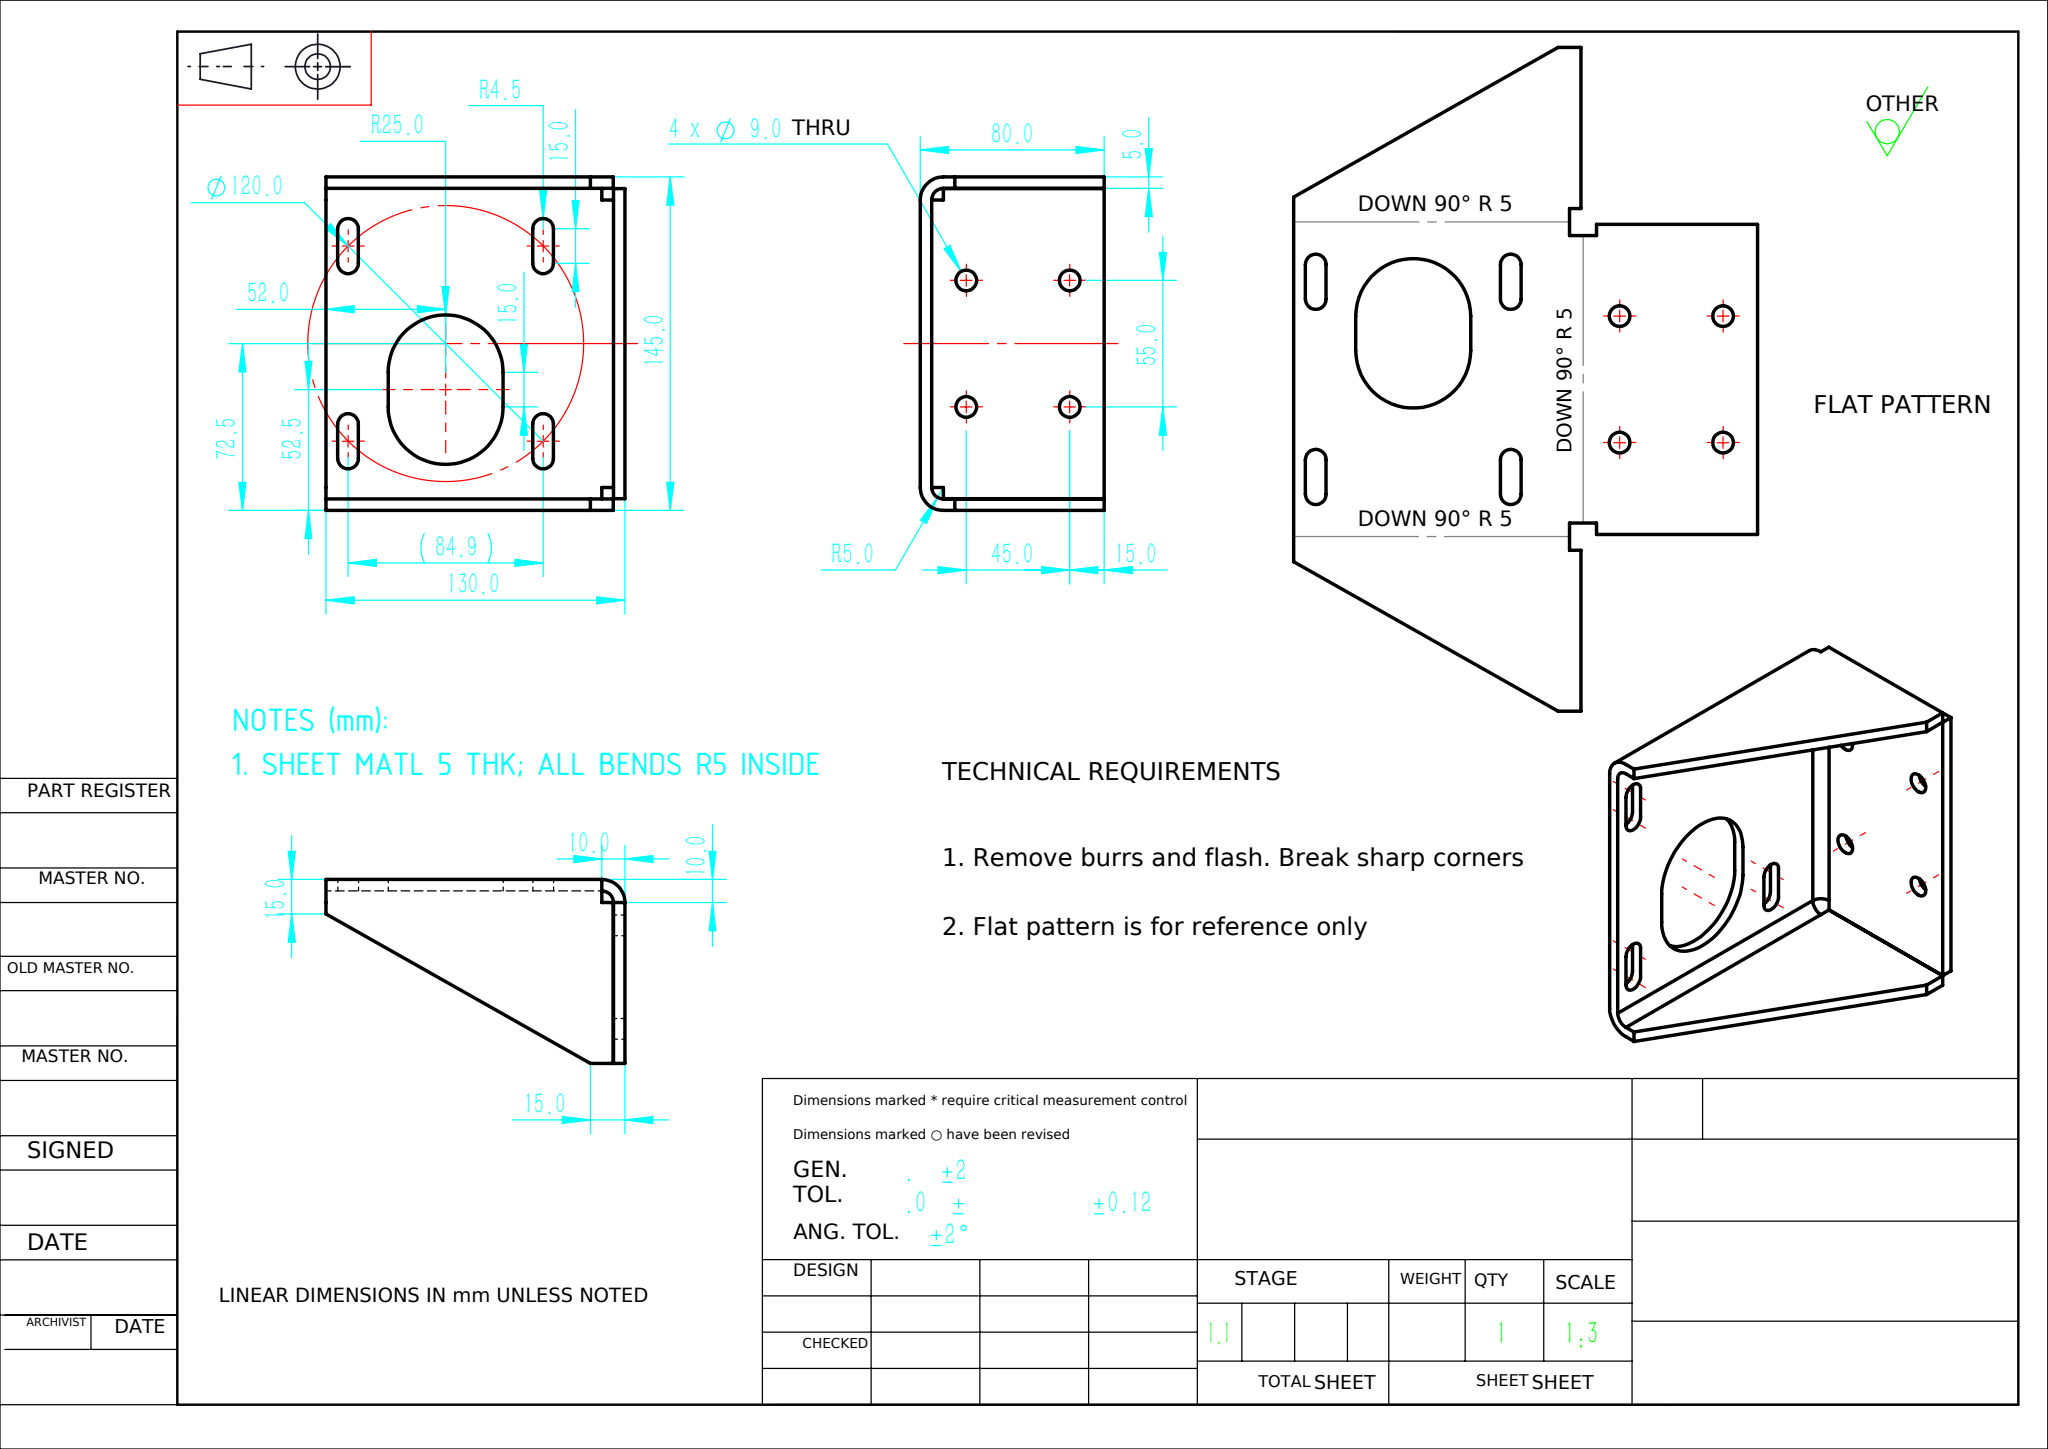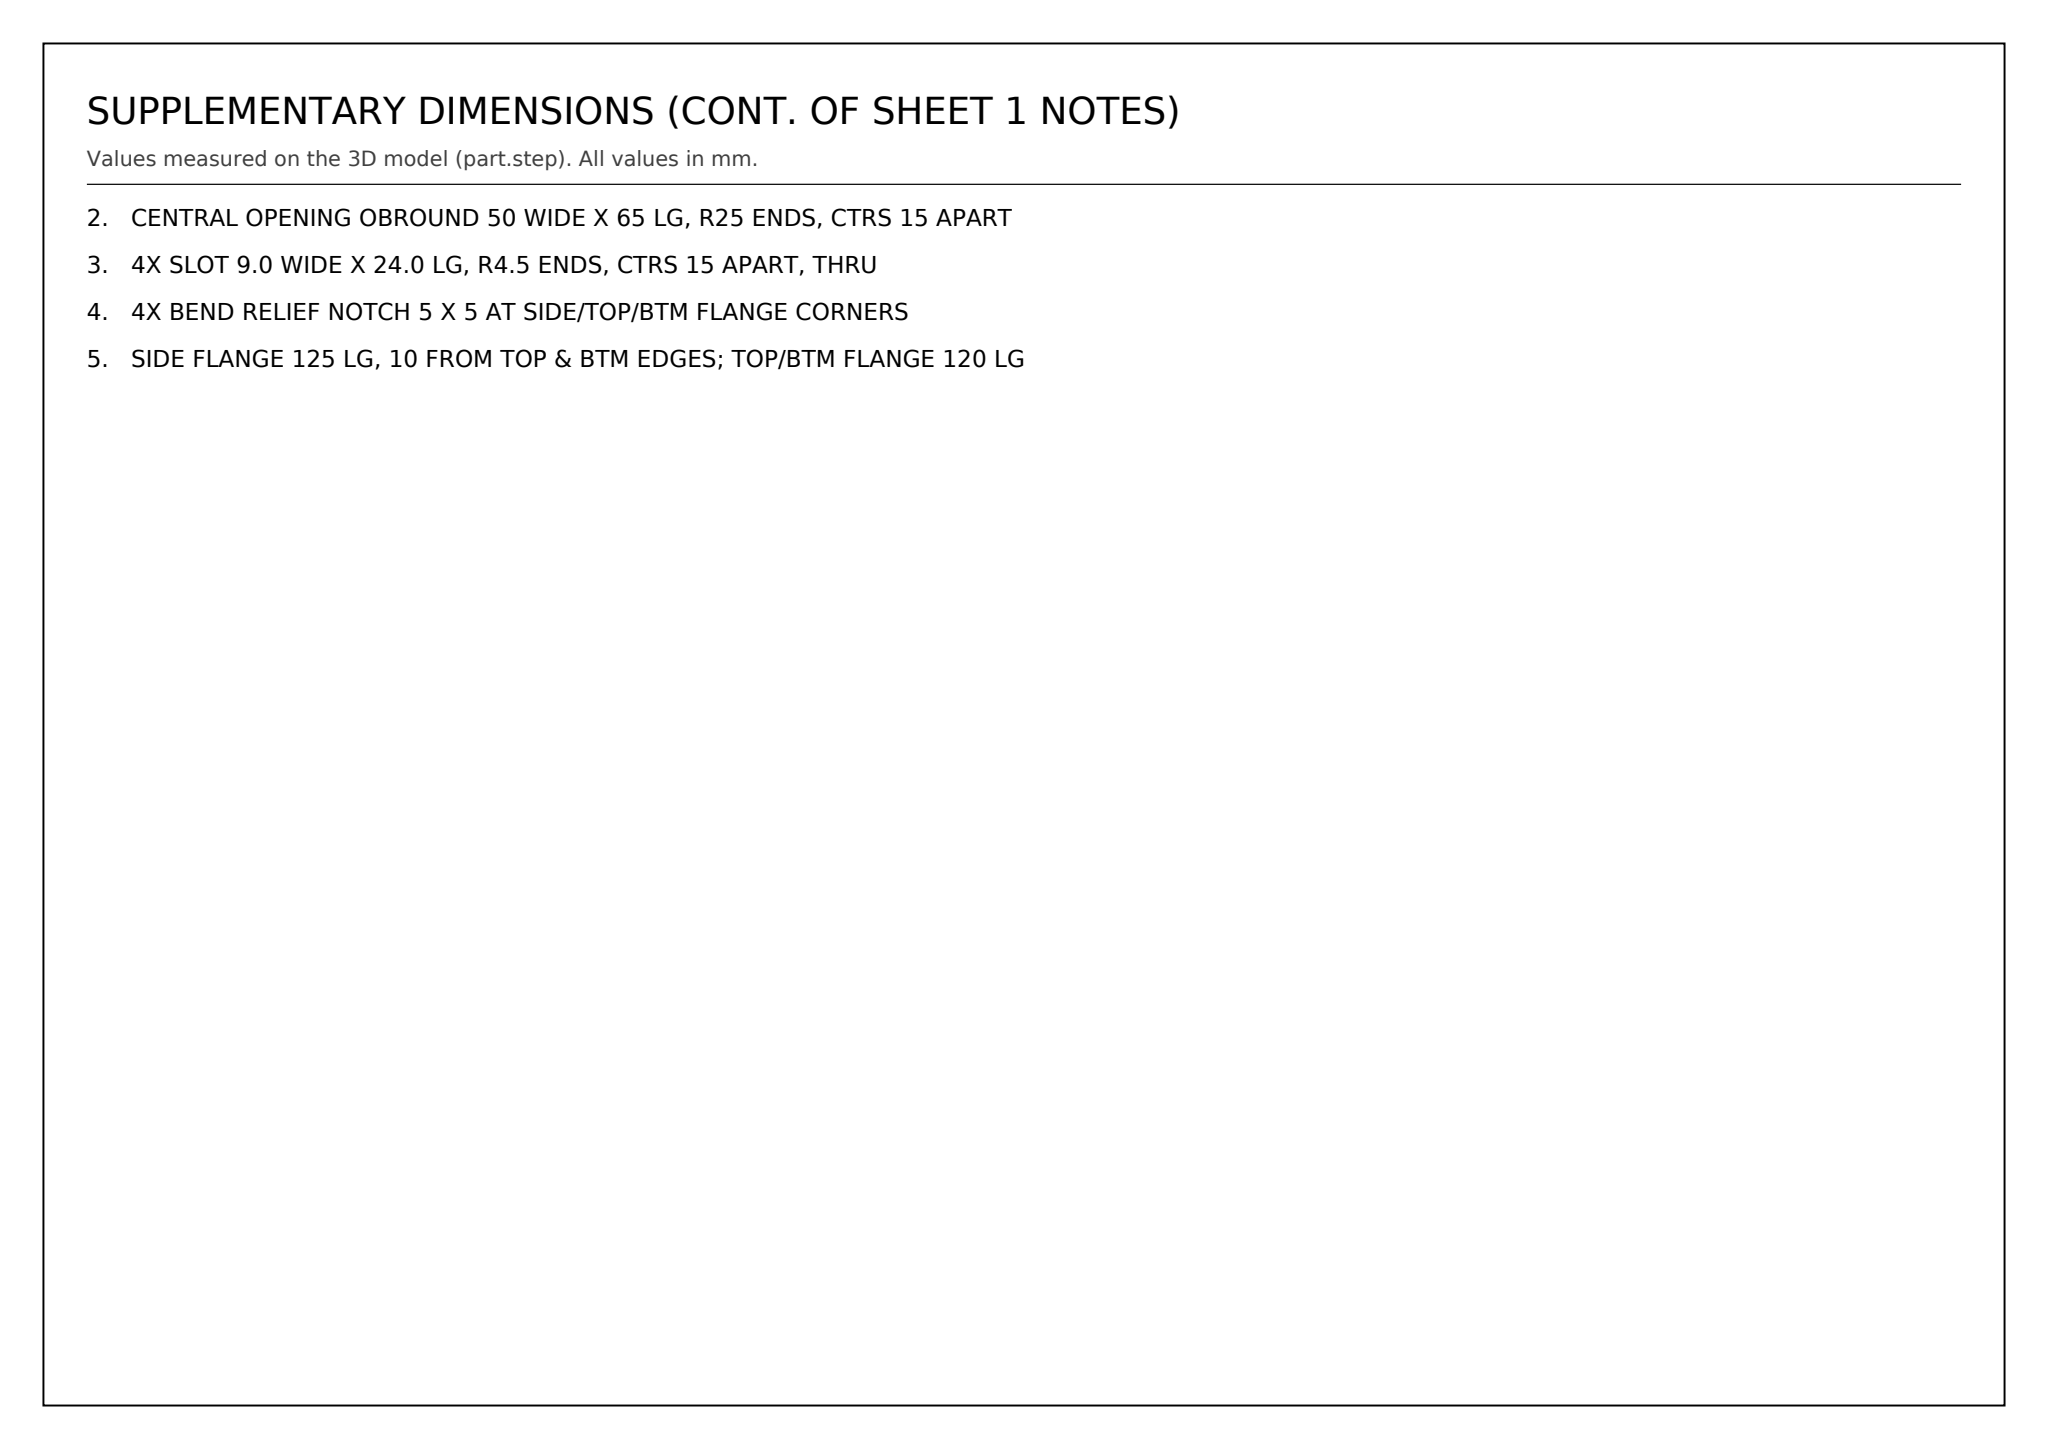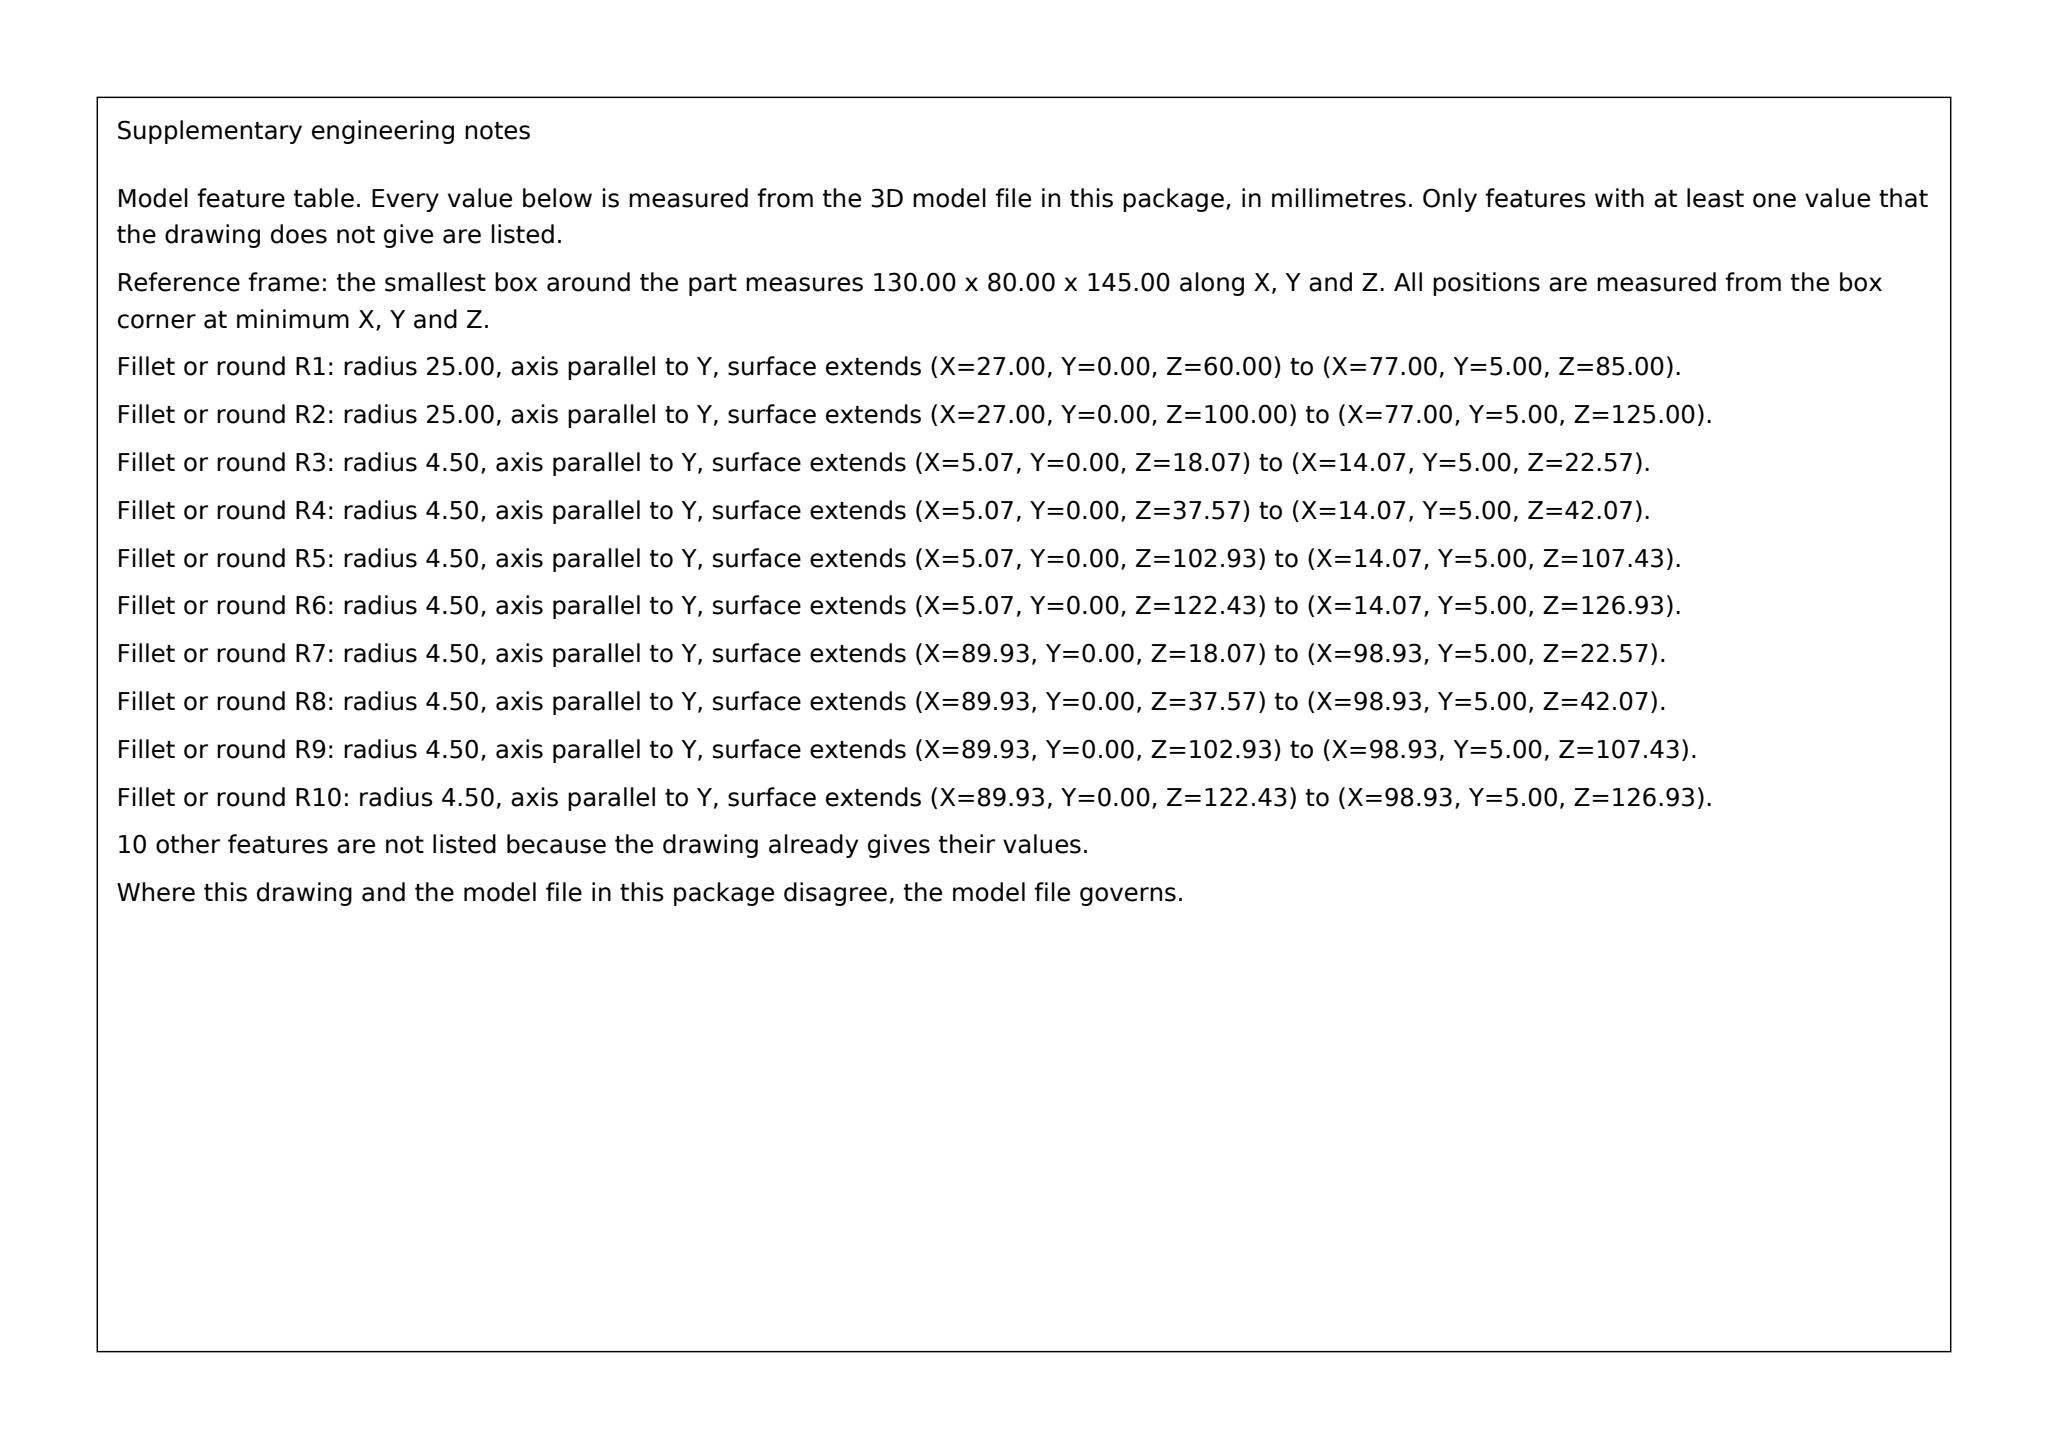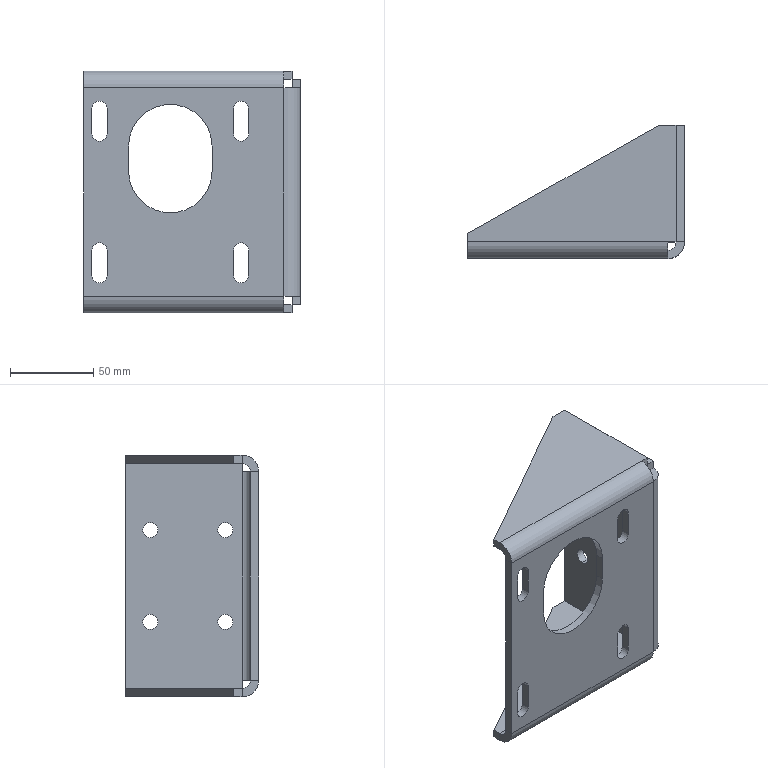Part | SolidWorks | mm | 1 solid | 64 faces | box 130 x 80 x 145 mm | volume 174964 mm3 | plane 40 | cylinder 24 | commonest cylinder face diameters 9 x16 20 x3 10 x3 50 x2
Drawing notes:
SHEET MATL 5 THK; ALL BENDS R5 INSIDE | from the solid: Planes y=0/5.0 and z=0/5.0; all hole cyls length 5.0
CENTRAL OPENING OBROUND 50 WIDE X 65 LG, R25 ENDS, CTRS 15 APART | from the solid: Two Ø50 y-axis cyls at (x52,z85) & (x52,z100), len 5.0
4X SLOT 9.0 WIDE X 24.0 LG, R4.5 ENDS, CTRS 15 APART, THRU | from the solid: Ø9 y-axis cyl pairs z22.57/37.57 & z107.43/122.43 at x9.57 & x94.43
4X BEND RELIEF NOTCH 5 X 5 AT SIDE/TOP/BTM FLANGE CORNERS | from the solid: x planes 120.0/124.93/125.0 and z planes 5.0/5.07/139.93/140.0 define 5x5 cut-outs at the 4 flange intersections
SIDE FLANGE 125 LG, 10 FROM TOP & BTM EDGES; TOP/BTM FLANGE 120 LG | from the solid: bend cyl dia10/20 axis z at x=120 len 125 (z 10-135); bend cyls dia10/20 axis x at z=10 & z=135 len 120 (x 0-120); bbox 130x80x145